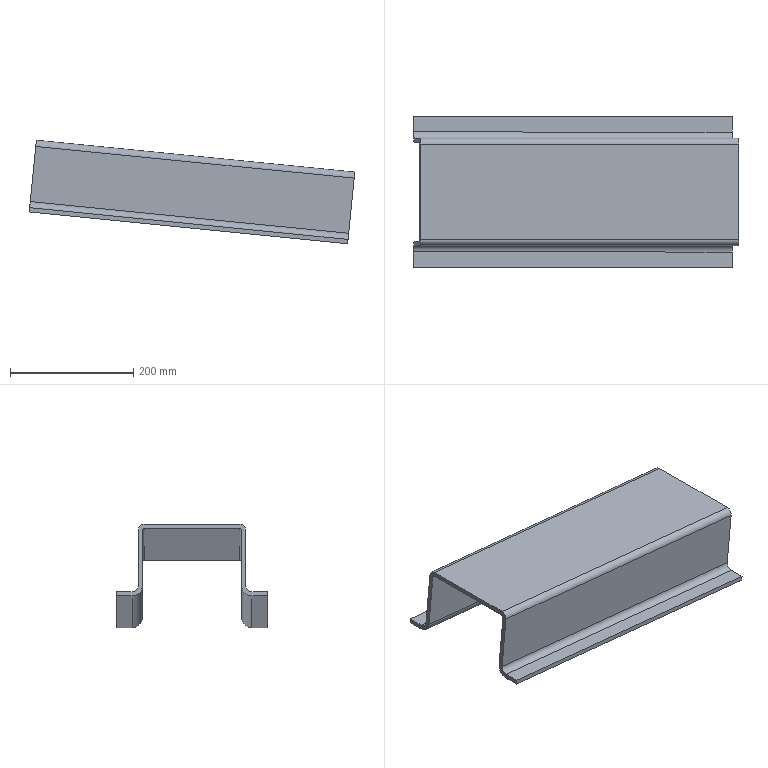Component | NX | MOVING_FRAME | 1 solid | 22 faces | volume 1630108 mm3 | plane 14 | cylinder 8 | commonest cylinder face diameters 20 x4 34 x2 6 x2